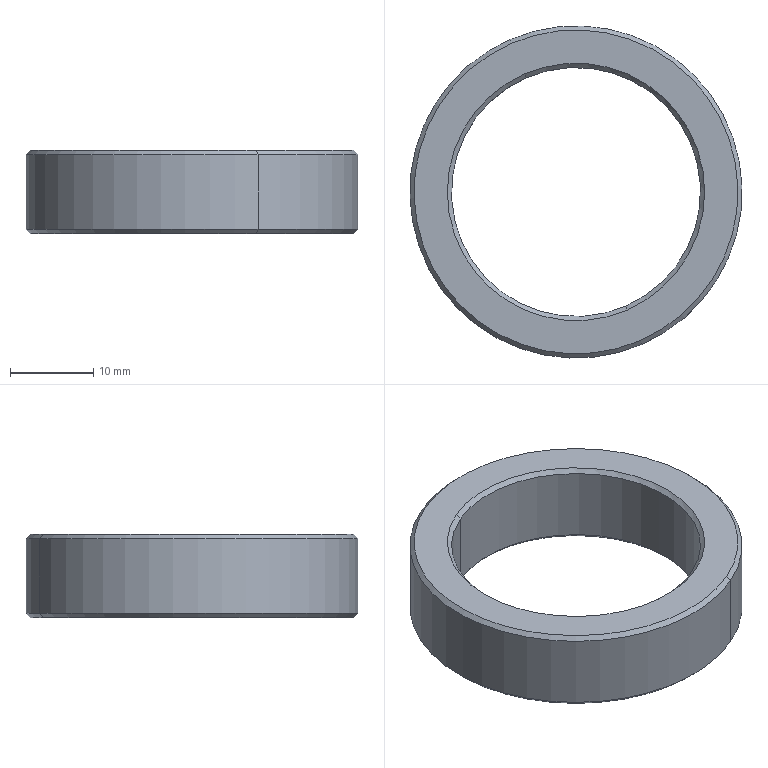Component | SolidWorks | Spacer30101-2 | 1 solid | 14 faces | box 40 x 40 x 10 mm | volume 5443 mm3 | cone 8 | cylinder 4 | plane 2 | commonest cylinder face diameters 30 x2 40 x2
build123d program:
from build123d import *

# Parameters (mm, degrees)
SKETCH1_R           = 20
SKETCH1_R_2         = 15
BOSS_EXTRUDE1_DEPTH = 10
CHAMFER1_SIZE       = 0.5


with BuildPart() as part:
    # Sketch1 → Boss-Extrude1 (new body)
    with BuildSketch(Plane(origin=(0, 0, 0), x_dir=(1, 0, 0), z_dir=(0, 1, 0))):
        with Locations(Location((0, 0, 0), (0, 0, 270))):
            Circle(SKETCH1_R)
        with Locations(Location((0, 0, 0), (0, 0, 270))):
            Circle(SKETCH1_R_2, mode=Mode.SUBTRACT)
    extrude(amount=BOSS_EXTRUDE1_DEPTH)

    # Chamfer1
    chamfer1_edges = [part.edges().sort_by_distance(p)[0] for p in [
        (0, 0, -20),
        (0, 10, -20),
        (0, 0, -15),
        (0, 10, -15),
    ]]
    chamfer(chamfer1_edges, length=CHAMFER1_SIZE)


solid = part.part

# Placed as in the assembly
solid = solid.moved(Location((-84.74, 20.354, 27), (90, 0, 0)))
STEP:
#1=COLOUR_RGB('',0.7922,0.8196,0.9333);
#2=FILL_AREA_STYLE_COLOUR('',#1);
#3=FILL_AREA_STYLE('',(#2));
#4=SURFACE_STYLE_FILL_AREA(#3);
#5=SURFACE_SIDE_STYLE('',(#4));
#6=SURFACE_STYLE_USAGE(.BOTH.,#5);
#7=PRESENTATION_STYLE_ASSIGNMENT((#6));
#8=CARTESIAN_POINT('',(-3.031,0.09688,1.063));
#9=VERTEX_POINT('',#8);
#10=CARTESIAN_POINT('',(-3.641,1.506,1.063));
#11=VERTEX_POINT('',#10);
#12=CARTESIAN_POINT('',(-3.336,0.8013,1.063));
#13=DIRECTION('',(-0.,-0.,-1.));
#14=DIRECTION('',(0.3975,-0.9176,-0.));
#15=AXIS2_PLACEMENT_3D('',#12,#13,#14);
#16=CIRCLE('',#15,0.7677);
#17=EDGE_CURVE('',#9,#11,#16,.T.);
#18=ORIENTED_EDGE('',*,*,#17,.F.);
#19=CARTESIAN_POINT('',(-3.023,0.07882,1.083));
#20=VERTEX_POINT('',#19);
#21=CARTESIAN_POINT('',(-3.031,0.09688,1.063));
#22=DIRECTION('',(0.2811,-0.6488,0.7071));
#23=VECTOR('',#22,39.37);
#24=LINE('',#21,#23);
#25=EDGE_CURVE('',#9,#20,#24,.T.);
#26=ORIENTED_EDGE('',*,*,#25,.T.);
#27=CARTESIAN_POINT('',(-3.649,1.524,1.083));
#28=VERTEX_POINT('',#27);
#29=CARTESIAN_POINT('',(-3.336,0.8013,1.083));
#30=DIRECTION('',(0.,0.,1.));
#31=DIRECTION('',(0.3975,-0.9176,-0.));
#32=AXIS2_PLACEMENT_3D('',#29,#30,#31);
#33=CIRCLE('',#32,0.7874);
#34=EDGE_CURVE('',#28,#20,#33,.T.);
#35=ORIENTED_EDGE('',*,*,#34,.F.);
#36=CARTESIAN_POINT('',(-3.641,1.506,1.063));
#37=DIRECTION('',(-0.2811,0.6488,0.7071));
#38=VECTOR('',#37,39.37);
#39=LINE('',#36,#38);
#40=EDGE_CURVE('',#11,#28,#39,.T.);
#41=ORIENTED_EDGE('',*,*,#40,.F.);
#42=EDGE_LOOP('',(#18,#26,#35,#41));
#43=FACE_OUTER_BOUND('',#42,.T.);
#44=CARTESIAN_POINT('',(-3.336,0.8013,1.063));
#45=DIRECTION('',(0.,0.,1.));
#46=DIRECTION('',(-0.3975,0.9176,0.));
#47=AXIS2_PLACEMENT_3D('',#44,#45,#46);
#48=CONICAL_SURFACE('',#47,0.7677,0.7854);
#49=ADVANCED_FACE('',(#43),#48,.T.);
#50=CARTESIAN_POINT('',(-3.571,1.343,1.083));
#51=VERTEX_POINT('',#50);
#52=CARTESIAN_POINT('',(-3.101,0.2594,1.083));
#53=VERTEX_POINT('',#52);
#54=CARTESIAN_POINT('',(-3.336,0.8013,1.083));
#55=DIRECTION('',(-0.,-0.,-1.));
#56=DIRECTION('',(0.3975,-0.9176,-0.));
#57=AXIS2_PLACEMENT_3D('',#54,#55,#56);
#58=CIRCLE('',#57,0.5906);
#59=EDGE_CURVE('',#51,#53,#58,.T.);
#60=ORIENTED_EDGE('',*,*,#59,.F.);
#61=CARTESIAN_POINT('',(-3.579,1.361,1.063));
#62=VERTEX_POINT('',#61);
#63=CARTESIAN_POINT('',(-3.571,1.343,1.083));
#64=DIRECTION('',(-0.2811,0.6488,-0.7071));
#65=VECTOR('',#64,39.37);
#66=LINE('',#63,#65);
#67=EDGE_CURVE('',#51,#62,#66,.T.);
#68=ORIENTED_EDGE('',*,*,#67,.T.);
#69=CARTESIAN_POINT('',(-3.094,0.2414,1.063));
#70=VERTEX_POINT('',#69);
#71=CARTESIAN_POINT('',(-3.336,0.8013,1.063));
#72=DIRECTION('',(0.,0.,1.));
#73=DIRECTION('',(0.3975,-0.9176,-0.));
#74=AXIS2_PLACEMENT_3D('',#71,#72,#73);
#75=CIRCLE('',#74,0.6102);
#76=EDGE_CURVE('',#70,#62,#75,.T.);
#77=ORIENTED_EDGE('',*,*,#76,.F.);
#78=CARTESIAN_POINT('',(-3.101,0.2594,1.083));
#79=DIRECTION('',(0.2811,-0.6488,-0.7071));
#80=VECTOR('',#79,39.37);
#81=LINE('',#78,#80);
#82=EDGE_CURVE('',#53,#70,#81,.T.);
#83=ORIENTED_EDGE('',*,*,#82,.F.);
#84=EDGE_LOOP('',(#60,#68,#77,#83));
#85=FACE_OUTER_BOUND('',#84,.T.);
#86=CARTESIAN_POINT('',(-3.336,0.8013,1.083));
#87=DIRECTION('',(-0.,-0.,-1.));
#88=DIRECTION('',(0.3975,-0.9176,-0.));
#89=AXIS2_PLACEMENT_3D('',#86,#87,#88);
#90=CONICAL_SURFACE('',#89,0.5906,0.7854);
#91=ADVANCED_FACE('',(#85),#90,.F.);
#92=CARTESIAN_POINT('',(-3.641,1.506,1.457));
#93=VERTEX_POINT('',#92);
#94=CARTESIAN_POINT('',(-3.031,0.09688,1.457));
#95=VERTEX_POINT('',#94);
#96=CARTESIAN_POINT('',(-3.336,0.8013,1.457));
#97=DIRECTION('',(0.,0.,1.));
#98=DIRECTION('',(0.3975,-0.9176,-0.));
#99=AXIS2_PLACEMENT_3D('',#96,#97,#98);
#100=CIRCLE('',#99,0.7677);
#101=EDGE_CURVE('',#93,#95,#100,.T.);
#102=ORIENTED_EDGE('',*,*,#101,.F.);
#103=CARTESIAN_POINT('',(-3.649,1.524,1.437));
#104=VERTEX_POINT('',#103);
#105=CARTESIAN_POINT('',(-3.649,1.524,1.437));
#106=DIRECTION('',(-0.2811,0.6488,-0.7071));
#107=VECTOR('',#106,39.37);
#108=LINE('',#105,#107);
#109=EDGE_CURVE('',#93,#104,#108,.T.);
#110=ORIENTED_EDGE('',*,*,#109,.T.);
#111=CARTESIAN_POINT('',(-3.023,0.07882,1.437));
#112=VERTEX_POINT('',#111);
#113=CARTESIAN_POINT('',(-3.336,0.8013,1.437));
#114=DIRECTION('',(-0.,-0.,-1.));
#115=DIRECTION('',(0.3975,-0.9176,-0.));
#116=AXIS2_PLACEMENT_3D('',#113,#114,#115);
#117=CIRCLE('',#116,0.7874);
#118=EDGE_CURVE('',#112,#104,#117,.T.);
#119=ORIENTED_EDGE('',*,*,#118,.F.);
#120=CARTESIAN_POINT('',(-3.023,0.07882,1.437));
#121=DIRECTION('',(0.2811,-0.6488,-0.7071));
#122=VECTOR('',#121,39.37);
#123=LINE('',#120,#122);
#124=EDGE_CURVE('',#95,#112,#123,.T.);
#125=ORIENTED_EDGE('',*,*,#124,.F.);
#126=EDGE_LOOP('',(#102,#110,#119,#125));
#127=FACE_OUTER_BOUND('',#126,.T.);
#128=CARTESIAN_POINT('',(-3.336,0.8013,1.437));
#129=DIRECTION('',(-0.,-0.,-1.));
#130=DIRECTION('',(0.3975,-0.9176,-0.));
#131=AXIS2_PLACEMENT_3D('',#128,#129,#130);
#132=CONICAL_SURFACE('',#131,0.7874,0.7854);
#133=ADVANCED_FACE('',(#127),#132,.T.);
#134=CARTESIAN_POINT('',(-3.101,0.2594,1.437));
#135=VERTEX_POINT('',#134);
#136=CARTESIAN_POINT('',(-3.571,1.343,1.437));
#137=VERTEX_POINT('',#136);
#138=CARTESIAN_POINT('',(-3.336,0.8013,1.437));
#139=DIRECTION('',(0.,0.,1.));
#140=DIRECTION('',(0.3975,-0.9176,-0.));
#141=AXIS2_PLACEMENT_3D('',#138,#139,#140);
#142=CIRCLE('',#141,0.5906);
#143=EDGE_CURVE('',#135,#137,#142,.T.);
#144=ORIENTED_EDGE('',*,*,#143,.F.);
#145=CARTESIAN_POINT('',(-3.094,0.2414,1.457));
#146=VERTEX_POINT('',#145);
#147=CARTESIAN_POINT('',(-3.094,0.2414,1.457));
#148=DIRECTION('',(0.2811,-0.6488,0.7071));
#149=VECTOR('',#148,39.37);
#150=LINE('',#147,#149);
#151=EDGE_CURVE('',#135,#146,#150,.T.);
#152=ORIENTED_EDGE('',*,*,#151,.T.);
#153=CARTESIAN_POINT('',(-3.579,1.361,1.457));
#154=VERTEX_POINT('',#153);
#155=CARTESIAN_POINT('',(-3.336,0.8013,1.457));
#156=DIRECTION('',(-0.,-0.,-1.));
#157=DIRECTION('',(0.3975,-0.9176,-0.));
#158=AXIS2_PLACEMENT_3D('',#155,#156,#157);
#159=CIRCLE('',#158,0.6102);
#160=EDGE_CURVE('',#154,#146,#159,.T.);
#161=ORIENTED_EDGE('',*,*,#160,.F.);
#162=CARTESIAN_POINT('',(-3.579,1.361,1.457));
#163=DIRECTION('',(-0.2811,0.6488,0.7071));
#164=VECTOR('',#163,39.37);
#165=LINE('',#162,#164);
#166=EDGE_CURVE('',#137,#154,#165,.T.);
#167=ORIENTED_EDGE('',*,*,#166,.F.);
#168=EDGE_LOOP('',(#144,#152,#161,#167));
#169=FACE_OUTER_BOUND('',#168,.T.);
#170=CARTESIAN_POINT('',(-3.336,0.8013,1.457));
#171=DIRECTION('',(0.,0.,1.));
#172=DIRECTION('',(-0.3975,0.9176,0.));
#173=AXIS2_PLACEMENT_3D('',#170,#171,#172);
#174=CONICAL_SURFACE('',#173,0.6102,0.7854);
#175=ADVANCED_FACE('',(#169),#174,.F.);
#176=ORIENTED_EDGE('',*,*,#59,.T.);
#177=CARTESIAN_POINT('',(-3.101,0.2594,1.063));
#178=DIRECTION('',(0.,0.,1.));
#179=VECTOR('',#178,39.37);
#180=LINE('',#177,#179);
#181=EDGE_CURVE('',#53,#135,#180,.T.);
#182=ORIENTED_EDGE('',*,*,#181,.T.);
#183=ORIENTED_EDGE('',*,*,#143,.T.);
#184=CARTESIAN_POINT('',(-3.571,1.343,1.063));
#185=DIRECTION('',(0.,0.,1.));
#186=VECTOR('',#185,39.37);
#187=LINE('',#184,#186);
#188=EDGE_CURVE('',#51,#137,#187,.T.);
#189=ORIENTED_EDGE('',*,*,#188,.F.);
#190=EDGE_LOOP('',(#176,#182,#183,#189));
#191=FACE_OUTER_BOUND('',#190,.T.);
#192=CARTESIAN_POINT('',(-3.336,0.8013,1.063));
#193=DIRECTION('',(0.,0.,1.));
#194=DIRECTION('',(-0.3975,0.9176,0.));
#195=AXIS2_PLACEMENT_3D('',#192,#193,#194);
#196=CYLINDRICAL_SURFACE('',#195,0.5906);
#197=ADVANCED_FACE('',(#191),#196,.F.);
#198=ORIENTED_EDGE('',*,*,#34,.T.);
#199=CARTESIAN_POINT('',(-3.023,0.07882,1.063));
#200=DIRECTION('',(0.,0.,1.));
#201=VECTOR('',#200,39.37);
#202=LINE('',#199,#201);
#203=EDGE_CURVE('',#20,#112,#202,.T.);
#204=ORIENTED_EDGE('',*,*,#203,.T.);
#205=ORIENTED_EDGE('',*,*,#118,.T.);
#206=CARTESIAN_POINT('',(-3.649,1.524,1.063));
#207=DIRECTION('',(0.,0.,1.));
#208=VECTOR('',#207,39.37);
#209=LINE('',#206,#208);
#210=EDGE_CURVE('',#28,#104,#209,.T.);
#211=ORIENTED_EDGE('',*,*,#210,.F.);
#212=EDGE_LOOP('',(#198,#204,#205,#211));
#213=FACE_OUTER_BOUND('',#212,.T.);
#214=CARTESIAN_POINT('',(-3.336,0.8013,1.063));
#215=DIRECTION('',(0.,0.,1.));
#216=DIRECTION('',(-0.3975,0.9176,0.));
#217=AXIS2_PLACEMENT_3D('',#214,#215,#216);
#218=CYLINDRICAL_SURFACE('',#217,0.7874);
#219=ADVANCED_FACE('',(#213),#218,.T.);
#220=ORIENTED_EDGE('',*,*,#76,.T.);
#221=CARTESIAN_POINT('',(-3.336,0.8013,1.063));
#222=DIRECTION('',(0.,0.,1.));
#223=DIRECTION('',(0.3975,-0.9176,-0.));
#224=AXIS2_PLACEMENT_3D('',#221,#222,#223);
#225=CIRCLE('',#224,0.6102);
#226=EDGE_CURVE('',#62,#70,#225,.T.);
#227=ORIENTED_EDGE('',*,*,#226,.T.);
#228=EDGE_LOOP('',(#220,#227));
#229=FACE_BOUND('',#228,.T.);
#230=CARTESIAN_POINT('',(-3.336,0.8013,1.063));
#231=DIRECTION('',(-0.,-0.,-1.));
#232=DIRECTION('',(0.3975,-0.9176,-0.));
#233=AXIS2_PLACEMENT_3D('',#230,#231,#232);
#234=CIRCLE('',#233,0.7677);
#235=EDGE_CURVE('',#11,#9,#234,.T.);
#236=ORIENTED_EDGE('',*,*,#235,.T.);
#237=ORIENTED_EDGE('',*,*,#17,.T.);
#238=EDGE_LOOP('',(#236,#237));
#239=FACE_OUTER_BOUND('',#238,.T.);
#240=CARTESIAN_POINT('',(-3.336,0.8013,1.063));
#241=DIRECTION('',(-0.,0.,-1.));
#242=DIRECTION('',(0.3975,-0.9176,-0.));
#243=AXIS2_PLACEMENT_3D('',#240,#241,#242);
#244=PLANE('',#243);
#245=ADVANCED_FACE('',(#229,#239),#244,.T.);
#246=ORIENTED_EDGE('',*,*,#160,.T.);
#247=CARTESIAN_POINT('',(-3.336,0.8013,1.457));
#248=DIRECTION('',(-0.,-0.,-1.));
#249=DIRECTION('',(0.3975,-0.9176,-0.));
#250=AXIS2_PLACEMENT_3D('',#247,#248,#249);
#251=CIRCLE('',#250,0.6102);
#252=EDGE_CURVE('',#146,#154,#251,.T.);
#253=ORIENTED_EDGE('',*,*,#252,.T.);
#254=EDGE_LOOP('',(#246,#253));
#255=FACE_BOUND('',#254,.T.);
#256=CARTESIAN_POINT('',(-3.336,0.8013,1.457));
#257=DIRECTION('',(0.,0.,1.));
#258=DIRECTION('',(0.3975,-0.9176,-0.));
#259=AXIS2_PLACEMENT_3D('',#256,#257,#258);
#260=CIRCLE('',#259,0.7677);
#261=EDGE_CURVE('',#95,#93,#260,.T.);
#262=ORIENTED_EDGE('',*,*,#261,.T.);
#263=ORIENTED_EDGE('',*,*,#101,.T.);
#264=EDGE_LOOP('',(#262,#263));
#265=FACE_OUTER_BOUND('',#264,.T.);
#266=CARTESIAN_POINT('',(-3.336,0.8013,1.457));
#267=DIRECTION('',(-0.,0.,-1.));
#268=DIRECTION('',(0.3975,-0.9176,-0.));
#269=AXIS2_PLACEMENT_3D('',#266,#267,#268);
#270=PLANE('',#269);
#271=ADVANCED_FACE('',(#255,#265),#270,.F.);
#272=ORIENTED_EDGE('',*,*,#203,.F.);
#273=CARTESIAN_POINT('',(-3.336,0.8013,1.083));
#274=DIRECTION('',(0.,0.,1.));
#275=DIRECTION('',(0.3975,-0.9176,-0.));
#276=AXIS2_PLACEMENT_3D('',#273,#274,#275);
#277=CIRCLE('',#276,0.7874);
#278=EDGE_CURVE('',#20,#28,#277,.T.);
#279=ORIENTED_EDGE('',*,*,#278,.T.);
#280=ORIENTED_EDGE('',*,*,#210,.T.);
#281=CARTESIAN_POINT('',(-3.336,0.8013,1.437));
#282=DIRECTION('',(-0.,-0.,-1.));
#283=DIRECTION('',(0.3975,-0.9176,-0.));
#284=AXIS2_PLACEMENT_3D('',#281,#282,#283);
#285=CIRCLE('',#284,0.7874);
#286=EDGE_CURVE('',#104,#112,#285,.T.);
#287=ORIENTED_EDGE('',*,*,#286,.T.);
#288=EDGE_LOOP('',(#272,#279,#280,#287));
#289=FACE_OUTER_BOUND('',#288,.T.);
#290=CARTESIAN_POINT('',(-3.336,0.8013,1.063));
#291=DIRECTION('',(0.,0.,1.));
#292=DIRECTION('',(-0.3975,0.9176,0.));
#293=AXIS2_PLACEMENT_3D('',#290,#291,#292);
#294=CYLINDRICAL_SURFACE('',#293,0.7874);
#295=ADVANCED_FACE('',(#289),#294,.T.);
#296=ORIENTED_EDGE('',*,*,#181,.F.);
#297=CARTESIAN_POINT('',(-3.336,0.8013,1.083));
#298=DIRECTION('',(-0.,-0.,-1.));
#299=DIRECTION('',(0.3975,-0.9176,-0.));
#300=AXIS2_PLACEMENT_3D('',#297,#298,#299);
#301=CIRCLE('',#300,0.5906);
#302=EDGE_CURVE('',#53,#51,#301,.T.);
#303=ORIENTED_EDGE('',*,*,#302,.T.);
#304=ORIENTED_EDGE('',*,*,#188,.T.);
#305=CARTESIAN_POINT('',(-3.336,0.8013,1.437));
#306=DIRECTION('',(0.,0.,1.));
#307=DIRECTION('',(0.3975,-0.9176,-0.));
#308=AXIS2_PLACEMENT_3D('',#305,#306,#307);
#309=CIRCLE('',#308,0.5906);
#310=EDGE_CURVE('',#137,#135,#309,.T.);
#311=ORIENTED_EDGE('',*,*,#310,.T.);
#312=EDGE_LOOP('',(#296,#303,#304,#311));
#313=FACE_OUTER_BOUND('',#312,.T.);
#314=CARTESIAN_POINT('',(-3.336,0.8013,1.063));
#315=DIRECTION('',(0.,0.,1.));
#316=DIRECTION('',(-0.3975,0.9176,0.));
#317=AXIS2_PLACEMENT_3D('',#314,#315,#316);
#318=CYLINDRICAL_SURFACE('',#317,0.5906);
#319=ADVANCED_FACE('',(#313),#318,.F.);
#320=ORIENTED_EDGE('',*,*,#151,.F.);
#321=ORIENTED_EDGE('',*,*,#310,.F.);
#322=ORIENTED_EDGE('',*,*,#166,.T.);
#323=ORIENTED_EDGE('',*,*,#252,.F.);
#324=EDGE_LOOP('',(#320,#321,#322,#323));
#325=FACE_OUTER_BOUND('',#324,.T.);
#326=CARTESIAN_POINT('',(-3.336,0.8013,1.457));
#327=DIRECTION('',(0.,0.,1.));
#328=DIRECTION('',(-0.3975,0.9176,0.));
#329=AXIS2_PLACEMENT_3D('',#326,#327,#328);
#330=CONICAL_SURFACE('',#329,0.6102,0.7854);
#331=ADVANCED_FACE('',(#325),#330,.F.);
#332=ORIENTED_EDGE('',*,*,#109,.F.);
#333=ORIENTED_EDGE('',*,*,#261,.F.);
#334=ORIENTED_EDGE('',*,*,#124,.T.);
#335=ORIENTED_EDGE('',*,*,#286,.F.);
#336=EDGE_LOOP('',(#332,#333,#334,#335));
#337=FACE_OUTER_BOUND('',#336,.T.);
#338=CARTESIAN_POINT('',(-3.336,0.8013,1.437));
#339=DIRECTION('',(-0.,-0.,-1.));
#340=DIRECTION('',(0.3975,-0.9176,-0.));
#341=AXIS2_PLACEMENT_3D('',#338,#339,#340);
#342=CONICAL_SURFACE('',#341,0.7874,0.7854);
#343=ADVANCED_FACE('',(#337),#342,.T.);
#344=ORIENTED_EDGE('',*,*,#67,.F.);
#345=ORIENTED_EDGE('',*,*,#302,.F.);
#346=ORIENTED_EDGE('',*,*,#82,.T.);
#347=ORIENTED_EDGE('',*,*,#226,.F.);
#348=EDGE_LOOP('',(#344,#345,#346,#347));
#349=FACE_OUTER_BOUND('',#348,.T.);
#350=CARTESIAN_POINT('',(-3.336,0.8013,1.083));
#351=DIRECTION('',(-0.,-0.,-1.));
#352=DIRECTION('',(0.3975,-0.9176,-0.));
#353=AXIS2_PLACEMENT_3D('',#350,#351,#352);
#354=CONICAL_SURFACE('',#353,0.5906,0.7854);
#355=ADVANCED_FACE('',(#349),#354,.F.);
#356=ORIENTED_EDGE('',*,*,#25,.F.);
#357=ORIENTED_EDGE('',*,*,#235,.F.);
#358=ORIENTED_EDGE('',*,*,#40,.T.);
#359=ORIENTED_EDGE('',*,*,#278,.F.);
#360=EDGE_LOOP('',(#356,#357,#358,#359));
#361=FACE_OUTER_BOUND('',#360,.T.);
#362=CARTESIAN_POINT('',(-3.336,0.8013,1.063));
#363=DIRECTION('',(0.,0.,1.));
#364=DIRECTION('',(-0.3975,0.9176,0.));
#365=AXIS2_PLACEMENT_3D('',#362,#363,#364);
#366=CONICAL_SURFACE('',#365,0.7677,0.7854);
#367=ADVANCED_FACE('',(#361),#366,.T.);
#368=CLOSED_SHELL('',(#49,#91,#133,#175,#197,#219,#245,#271,#295,#319,#331,#343,#355,#367));
#369=MANIFOLD_SOLID_BREP('',#368);
#370=STYLED_ITEM('',(#7),#369);
#371=(LENGTH_UNIT()NAMED_UNIT(*)SI_UNIT($,.METRE.));
#372=LENGTH_MEASURE_WITH_UNIT(LENGTH_MEASURE(0.0254),#371);
#373=DIMENSIONAL_EXPONENTS(1.,0.,0.,0.,0.,0.,0.);
#374=(CONVERSION_BASED_UNIT('',#372)LENGTH_UNIT()NAMED_UNIT(#373));
#375=UNCERTAINTY_MEASURE_WITH_UNIT(LENGTH_MEASURE(0.00001),#374,'','');
#376=(NAMED_UNIT(*)PLANE_ANGLE_UNIT()SI_UNIT($,.RADIAN.));
#377=(NAMED_UNIT(*)SI_UNIT($,.STERADIAN.)SOLID_ANGLE_UNIT());
#378=(GEOMETRIC_REPRESENTATION_CONTEXT(3)GLOBAL_UNCERTAINTY_ASSIGNED_CONTEXT((#375))GLOBAL_UNIT_ASSIGNED_CONTEXT((#374,#376,#377))REPRESENTATION_CONTEXT('',''));
#379=MECHANICAL_DESIGN_GEOMETRIC_PRESENTATION_REPRESENTATION('',(#370),#378);
#380=PRESENTATION_LAYER_ASSIGNMENT('','',(#370));
#381=CARTESIAN_POINT('',(0.,0.,0.));
#382=DIRECTION('',(0.,0.,1.));
#383=DIRECTION('',(1.,0.,0.));
#384=AXIS2_PLACEMENT_3D('',#381,#382,#383);
#385=(LENGTH_UNIT()NAMED_UNIT(*)SI_UNIT($,.METRE.));
#386=LENGTH_MEASURE_WITH_UNIT(LENGTH_MEASURE(0.0254),#385);
#387=DIMENSIONAL_EXPONENTS(1.,0.,0.,0.,0.,0.,0.);
#388=(CONVERSION_BASED_UNIT('',#386)LENGTH_UNIT()NAMED_UNIT(#387));
#389=UNCERTAINTY_MEASURE_WITH_UNIT(LENGTH_MEASURE(0.00001),#388,'','');
#390=(NAMED_UNIT(*)PLANE_ANGLE_UNIT()SI_UNIT($,.RADIAN.));
#391=(NAMED_UNIT(*)SI_UNIT($,.STERADIAN.)SOLID_ANGLE_UNIT());
#392=(GEOMETRIC_REPRESENTATION_CONTEXT(3)GLOBAL_UNCERTAINTY_ASSIGNED_CONTEXT((#389))GLOBAL_UNIT_ASSIGNED_CONTEXT((#388,#390,#391))REPRESENTATION_CONTEXT('',''));
#393=ADVANCED_BREP_SHAPE_REPRESENTATION('',(#369,#384),#392);